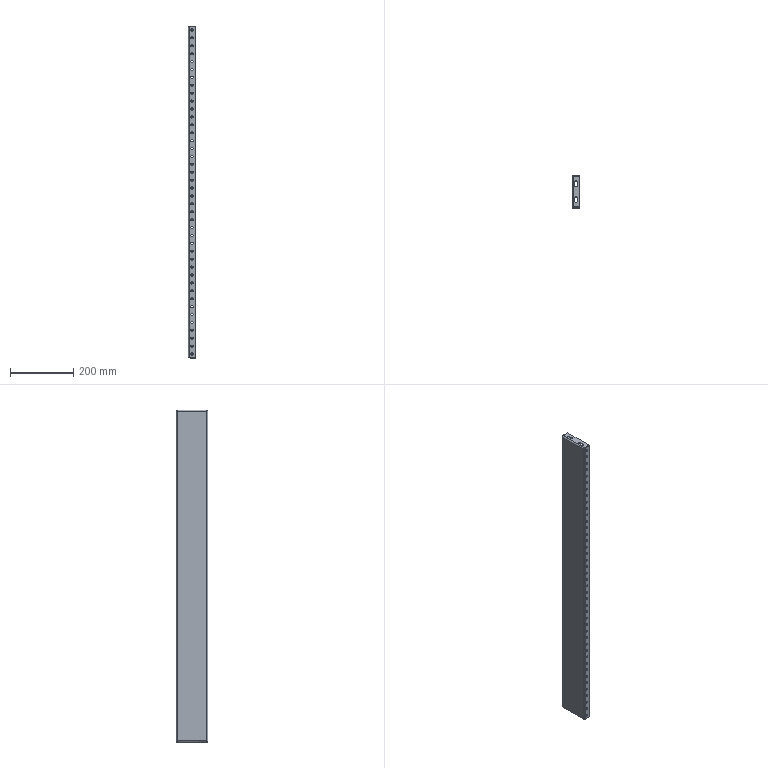Component | SolidWorks | MountingColumn-2 | 1 solid | 226 faces | volume 301886 mm3 | cylinder 188 | plane 30 | spline 8 | commonest cylinder face diameters 7 x180 8 x4 4 x4